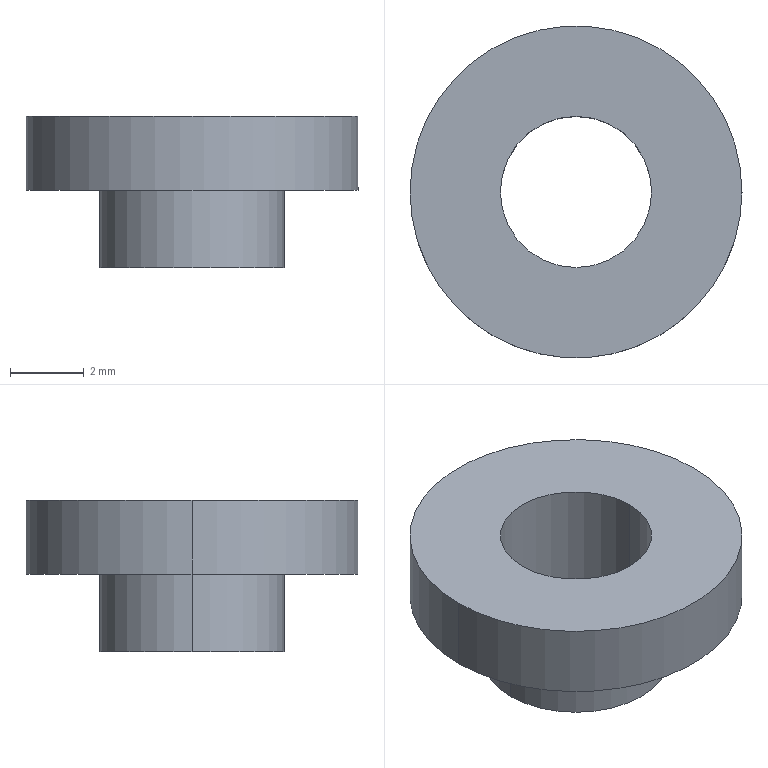Component | SolidWorks | BSH3-02-00ARubberBlankingAssembly2-1_BSH3-02-09Gasket-1 | 1 solid | 9 faces | box 9 x 9 x 4.1 mm | volume 114 mm3 | cylinder 6 | plane 3 | commonest cylinder face diameters 9 x2 5 x2 4.1 x2
build123d program:
from build123d import *


with BuildPart() as part:
    # Sketch1 → Revolve1 (revolve)
    with BuildSketch(Plane.XY, mode=Mode.PRIVATE) as revolve1_sk:
        Polygon((2.05, 0), (2.05, 4.1), (2.5, 4.1), (2.5, 2), (4.5, 2), (4.5, 0), align=None)
    revolve(revolve1_sk.sketch.rotate(Axis((0, 0, 0), (0, 1, 0)), 90), axis=Axis((0, 0, 0), (0, 1, 0)))


solid = part.part

# Placed as in the assembly
solid = solid.moved(Location((85.629, 20.762, -3.139), (-90, 0, 0)))
STEP:
#1=CARTESIAN_POINT('',(3.548,0.8174,-0.2023));
#2=VERTEX_POINT('',#1);
#3=CARTESIAN_POINT('',(3.194,0.8174,-0.2023));
#4=VERTEX_POINT('',#3);
#5=CARTESIAN_POINT('',(3.371,0.8174,-0.2023));
#6=DIRECTION('',(0.,0.,1.));
#7=DIRECTION('',(1.,0.,0.));
#8=AXIS2_PLACEMENT_3D('',#5,#6,#7);
#9=CIRCLE('',#8,0.1772);
#10=EDGE_CURVE('',#2,#4,#9,.T.);
#11=ORIENTED_EDGE('',*,*,#10,.T.);
#12=CARTESIAN_POINT('',(3.194,0.8174,-0.1236));
#13=VERTEX_POINT('',#12);
#14=CARTESIAN_POINT('',(3.194,0.8174,-0.1236));
#15=DIRECTION('',(0.,0.,1.));
#16=VECTOR('',#15,39.37);
#17=LINE('',#14,#16);
#18=EDGE_CURVE('',#4,#13,#17,.T.);
#19=ORIENTED_EDGE('',*,*,#18,.T.);
#20=CARTESIAN_POINT('',(3.548,0.8174,-0.1236));
#21=VERTEX_POINT('',#20);
#22=CARTESIAN_POINT('',(3.371,0.8174,-0.1236));
#23=DIRECTION('',(0.,0.,1.));
#24=DIRECTION('',(1.,0.,0.));
#25=AXIS2_PLACEMENT_3D('',#22,#23,#24);
#26=CIRCLE('',#25,0.1772);
#27=EDGE_CURVE('',#21,#13,#26,.T.);
#28=ORIENTED_EDGE('',*,*,#27,.F.);
#29=CARTESIAN_POINT('',(3.548,0.8174,-0.1236));
#30=DIRECTION('',(0.,0.,1.));
#31=VECTOR('',#30,39.37);
#32=LINE('',#29,#31);
#33=EDGE_CURVE('',#2,#21,#32,.T.);
#34=ORIENTED_EDGE('',*,*,#33,.F.);
#35=EDGE_LOOP('',(#11,#19,#28,#34));
#36=FACE_OUTER_BOUND('',#35,.T.);
#37=CARTESIAN_POINT('',(3.371,0.8174,-0.1236));
#38=DIRECTION('',(0.,0.,1.));
#39=DIRECTION('',(1.,0.,0.));
#40=AXIS2_PLACEMENT_3D('',#37,#38,#39);
#41=CYLINDRICAL_SURFACE('',#40,0.1772);
#42=ADVANCED_FACE('',(#36),#41,.T.);
#43=CARTESIAN_POINT('',(3.47,0.8174,-0.285));
#44=VERTEX_POINT('',#43);
#45=CARTESIAN_POINT('',(3.273,0.8174,-0.285));
#46=VERTEX_POINT('',#45);
#47=CARTESIAN_POINT('',(3.371,0.8174,-0.285));
#48=DIRECTION('',(0.,0.,1.));
#49=DIRECTION('',(1.,0.,0.));
#50=AXIS2_PLACEMENT_3D('',#47,#48,#49);
#51=CIRCLE('',#50,0.09843);
#52=EDGE_CURVE('',#44,#46,#51,.T.);
#53=ORIENTED_EDGE('',*,*,#52,.T.);
#54=CARTESIAN_POINT('',(3.273,0.8174,-0.2023));
#55=VERTEX_POINT('',#54);
#56=CARTESIAN_POINT('',(3.273,0.8174,-0.1236));
#57=DIRECTION('',(0.,0.,1.));
#58=VECTOR('',#57,39.37);
#59=LINE('',#56,#58);
#60=EDGE_CURVE('',#46,#55,#59,.T.);
#61=ORIENTED_EDGE('',*,*,#60,.T.);
#62=CARTESIAN_POINT('',(3.47,0.8174,-0.2023));
#63=VERTEX_POINT('',#62);
#64=CARTESIAN_POINT('',(3.371,0.8174,-0.2023));
#65=DIRECTION('',(0.,0.,1.));
#66=DIRECTION('',(1.,0.,0.));
#67=AXIS2_PLACEMENT_3D('',#64,#65,#66);
#68=CIRCLE('',#67,0.09843);
#69=EDGE_CURVE('',#63,#55,#68,.T.);
#70=ORIENTED_EDGE('',*,*,#69,.F.);
#71=CARTESIAN_POINT('',(3.47,0.8174,-0.1236));
#72=DIRECTION('',(0.,0.,1.));
#73=VECTOR('',#72,39.37);
#74=LINE('',#71,#73);
#75=EDGE_CURVE('',#44,#63,#74,.T.);
#76=ORIENTED_EDGE('',*,*,#75,.F.);
#77=EDGE_LOOP('',(#53,#61,#70,#76));
#78=FACE_OUTER_BOUND('',#77,.T.);
#79=CARTESIAN_POINT('',(3.371,0.8174,-0.1236));
#80=DIRECTION('',(0.,0.,1.));
#81=DIRECTION('',(1.,0.,0.));
#82=AXIS2_PLACEMENT_3D('',#79,#80,#81);
#83=CYLINDRICAL_SURFACE('',#82,0.09843);
#84=ADVANCED_FACE('',(#78),#83,.T.);
#85=CARTESIAN_POINT('',(3.291,0.8174,-0.285));
#86=VERTEX_POINT('',#85);
#87=CARTESIAN_POINT('',(3.452,0.8174,-0.285));
#88=VERTEX_POINT('',#87);
#89=CARTESIAN_POINT('',(3.371,0.8174,-0.285));
#90=DIRECTION('',(0.,0.,1.));
#91=DIRECTION('',(1.,0.,0.));
#92=AXIS2_PLACEMENT_3D('',#89,#90,#91);
#93=CIRCLE('',#92,0.08071);
#94=EDGE_CURVE('',#86,#88,#93,.T.);
#95=ORIENTED_EDGE('',*,*,#94,.F.);
#96=CARTESIAN_POINT('',(3.291,0.8174,-0.1236));
#97=VERTEX_POINT('',#96);
#98=CARTESIAN_POINT('',(3.291,0.8174,-0.1236));
#99=DIRECTION('',(0.,0.,1.));
#100=VECTOR('',#99,39.37);
#101=LINE('',#98,#100);
#102=EDGE_CURVE('',#86,#97,#101,.T.);
#103=ORIENTED_EDGE('',*,*,#102,.T.);
#104=CARTESIAN_POINT('',(3.452,0.8174,-0.1236));
#105=VERTEX_POINT('',#104);
#106=CARTESIAN_POINT('',(3.371,0.8174,-0.1236));
#107=DIRECTION('',(0.,0.,1.));
#108=DIRECTION('',(1.,0.,0.));
#109=AXIS2_PLACEMENT_3D('',#106,#107,#108);
#110=CIRCLE('',#109,0.08071);
#111=EDGE_CURVE('',#97,#105,#110,.T.);
#112=ORIENTED_EDGE('',*,*,#111,.T.);
#113=CARTESIAN_POINT('',(3.452,0.8174,-0.1236));
#114=DIRECTION('',(0.,0.,1.));
#115=VECTOR('',#114,39.37);
#116=LINE('',#113,#115);
#117=EDGE_CURVE('',#88,#105,#116,.T.);
#118=ORIENTED_EDGE('',*,*,#117,.F.);
#119=EDGE_LOOP('',(#95,#103,#112,#118));
#120=FACE_OUTER_BOUND('',#119,.T.);
#121=CARTESIAN_POINT('',(3.371,0.8174,-0.1236));
#122=DIRECTION('',(0.,0.,1.));
#123=DIRECTION('',(1.,0.,0.));
#124=AXIS2_PLACEMENT_3D('',#121,#122,#123);
#125=CYLINDRICAL_SURFACE('',#124,0.08071);
#126=ADVANCED_FACE('',(#120),#125,.F.);
#127=ORIENTED_EDGE('',*,*,#27,.T.);
#128=CARTESIAN_POINT('',(3.371,0.8174,-0.1236));
#129=DIRECTION('',(0.,0.,1.));
#130=DIRECTION('',(1.,0.,0.));
#131=AXIS2_PLACEMENT_3D('',#128,#129,#130);
#132=CIRCLE('',#131,0.1772);
#133=EDGE_CURVE('',#13,#21,#132,.T.);
#134=ORIENTED_EDGE('',*,*,#133,.T.);
#135=EDGE_LOOP('',(#127,#134));
#136=FACE_OUTER_BOUND('',#135,.T.);
#137=CARTESIAN_POINT('',(3.371,0.8174,-0.1236));
#138=DIRECTION('',(0.,0.,1.));
#139=DIRECTION('',(1.,0.,0.));
#140=AXIS2_PLACEMENT_3D('',#137,#138,#139);
#141=CIRCLE('',#140,0.08071);
#142=EDGE_CURVE('',#105,#97,#141,.T.);
#143=ORIENTED_EDGE('',*,*,#142,.F.);
#144=ORIENTED_EDGE('',*,*,#111,.F.);
#145=EDGE_LOOP('',(#143,#144));
#146=FACE_BOUND('',#145,.T.);
#147=CARTESIAN_POINT('',(3.371,0.9946,-0.1236));
#148=DIRECTION('',(0.,0.,1.));
#149=DIRECTION('',(1.,0.,-0.));
#150=AXIS2_PLACEMENT_3D('',#147,#148,#149);
#151=PLANE('',#150);
#152=ADVANCED_FACE('',(#136,#146),#151,.T.);
#153=ORIENTED_EDGE('',*,*,#102,.F.);
#154=CARTESIAN_POINT('',(3.371,0.8174,-0.285));
#155=DIRECTION('',(0.,0.,1.));
#156=DIRECTION('',(1.,0.,0.));
#157=AXIS2_PLACEMENT_3D('',#154,#155,#156);
#158=CIRCLE('',#157,0.08071);
#159=EDGE_CURVE('',#88,#86,#158,.T.);
#160=ORIENTED_EDGE('',*,*,#159,.F.);
#161=ORIENTED_EDGE('',*,*,#117,.T.);
#162=ORIENTED_EDGE('',*,*,#142,.T.);
#163=EDGE_LOOP('',(#153,#160,#161,#162));
#164=FACE_OUTER_BOUND('',#163,.T.);
#165=CARTESIAN_POINT('',(3.371,0.8174,-0.1236));
#166=DIRECTION('',(0.,0.,1.));
#167=DIRECTION('',(1.,0.,0.));
#168=AXIS2_PLACEMENT_3D('',#165,#166,#167);
#169=CYLINDRICAL_SURFACE('',#168,0.08071);
#170=ADVANCED_FACE('',(#164),#169,.F.);
#171=ORIENTED_EDGE('',*,*,#159,.T.);
#172=ORIENTED_EDGE('',*,*,#94,.T.);
#173=EDGE_LOOP('',(#171,#172));
#174=FACE_BOUND('',#173,.T.);
#175=ORIENTED_EDGE('',*,*,#52,.F.);
#176=CARTESIAN_POINT('',(3.371,0.8174,-0.285));
#177=DIRECTION('',(0.,0.,1.));
#178=DIRECTION('',(1.,0.,0.));
#179=AXIS2_PLACEMENT_3D('',#176,#177,#178);
#180=CIRCLE('',#179,0.09843);
#181=EDGE_CURVE('',#46,#44,#180,.T.);
#182=ORIENTED_EDGE('',*,*,#181,.F.);
#183=EDGE_LOOP('',(#175,#182));
#184=FACE_OUTER_BOUND('',#183,.T.);
#185=CARTESIAN_POINT('',(3.371,0.8981,-0.285));
#186=DIRECTION('',(-0.,-0.,-1.));
#187=DIRECTION('',(-1.,-0.,0.));
#188=AXIS2_PLACEMENT_3D('',#185,#186,#187);
#189=PLANE('',#188);
#190=ADVANCED_FACE('',(#174,#184),#189,.T.);
#191=ORIENTED_EDGE('',*,*,#60,.F.);
#192=ORIENTED_EDGE('',*,*,#181,.T.);
#193=ORIENTED_EDGE('',*,*,#75,.T.);
#194=CARTESIAN_POINT('',(3.371,0.8174,-0.2023));
#195=DIRECTION('',(0.,0.,1.));
#196=DIRECTION('',(1.,0.,0.));
#197=AXIS2_PLACEMENT_3D('',#194,#195,#196);
#198=CIRCLE('',#197,0.09843);
#199=EDGE_CURVE('',#55,#63,#198,.T.);
#200=ORIENTED_EDGE('',*,*,#199,.F.);
#201=EDGE_LOOP('',(#191,#192,#193,#200));
#202=FACE_OUTER_BOUND('',#201,.T.);
#203=CARTESIAN_POINT('',(3.371,0.8174,-0.1236));
#204=DIRECTION('',(0.,0.,1.));
#205=DIRECTION('',(1.,0.,0.));
#206=AXIS2_PLACEMENT_3D('',#203,#204,#205);
#207=CYLINDRICAL_SURFACE('',#206,0.09843);
#208=ADVANCED_FACE('',(#202),#207,.T.);
#209=ORIENTED_EDGE('',*,*,#69,.T.);
#210=ORIENTED_EDGE('',*,*,#199,.T.);
#211=EDGE_LOOP('',(#209,#210));
#212=FACE_BOUND('',#211,.T.);
#213=ORIENTED_EDGE('',*,*,#10,.F.);
#214=CARTESIAN_POINT('',(3.371,0.8174,-0.2023));
#215=DIRECTION('',(0.,0.,1.));
#216=DIRECTION('',(1.,0.,0.));
#217=AXIS2_PLACEMENT_3D('',#214,#215,#216);
#218=CIRCLE('',#217,0.1772);
#219=EDGE_CURVE('',#4,#2,#218,.T.);
#220=ORIENTED_EDGE('',*,*,#219,.F.);
#221=EDGE_LOOP('',(#213,#220));
#222=FACE_OUTER_BOUND('',#221,.T.);
#223=CARTESIAN_POINT('',(3.371,0.9158,-0.2023));
#224=DIRECTION('',(-0.,-0.,-1.));
#225=DIRECTION('',(-1.,-0.,0.));
#226=AXIS2_PLACEMENT_3D('',#223,#224,#225);
#227=PLANE('',#226);
#228=ADVANCED_FACE('',(#212,#222),#227,.T.);
#229=ORIENTED_EDGE('',*,*,#18,.F.);
#230=ORIENTED_EDGE('',*,*,#219,.T.);
#231=ORIENTED_EDGE('',*,*,#33,.T.);
#232=ORIENTED_EDGE('',*,*,#133,.F.);
#233=EDGE_LOOP('',(#229,#230,#231,#232));
#234=FACE_OUTER_BOUND('',#233,.T.);
#235=CARTESIAN_POINT('',(3.371,0.8174,-0.1236));
#236=DIRECTION('',(0.,0.,1.));
#237=DIRECTION('',(1.,0.,0.));
#238=AXIS2_PLACEMENT_3D('',#235,#236,#237);
#239=CYLINDRICAL_SURFACE('',#238,0.1772);
#240=ADVANCED_FACE('',(#234),#239,.T.);
#241=CLOSED_SHELL('',(#42,#84,#126,#152,#170,#190,#208,#228,#240));
#242=MANIFOLD_SOLID_BREP('',#241);
#243=CARTESIAN_POINT('',(0.,0.,0.));
#244=DIRECTION('',(0.,0.,1.));
#245=DIRECTION('',(1.,0.,0.));
#246=AXIS2_PLACEMENT_3D('',#243,#244,#245);
#247=(LENGTH_UNIT()NAMED_UNIT(*)SI_UNIT($,.METRE.));
#248=LENGTH_MEASURE_WITH_UNIT(LENGTH_MEASURE(0.0254),#247);
#249=DIMENSIONAL_EXPONENTS(1.,0.,0.,0.,0.,0.,0.);
#250=(CONVERSION_BASED_UNIT('',#248)LENGTH_UNIT()NAMED_UNIT(#249));
#251=UNCERTAINTY_MEASURE_WITH_UNIT(LENGTH_MEASURE(0.00001),#250,'','');
#252=(NAMED_UNIT(*)PLANE_ANGLE_UNIT()SI_UNIT($,.RADIAN.));
#253=(NAMED_UNIT(*)SI_UNIT($,.STERADIAN.)SOLID_ANGLE_UNIT());
#254=(GEOMETRIC_REPRESENTATION_CONTEXT(3)GLOBAL_UNCERTAINTY_ASSIGNED_CONTEXT((#251))GLOBAL_UNIT_ASSIGNED_CONTEXT((#250,#252,#253))REPRESENTATION_CONTEXT('',''));
#255=ADVANCED_BREP_SHAPE_REPRESENTATION('',(#242,#246),#254);
#256=COLOUR_RGB('',0.7922,0.8196,0.9333);
#257=FILL_AREA_STYLE_COLOUR('',#256);
#258=FILL_AREA_STYLE('',(#257));
#259=SURFACE_STYLE_FILL_AREA(#258);
#260=SURFACE_SIDE_STYLE('',(#259));
#261=SURFACE_STYLE_USAGE(.BOTH.,#260);
#262=PRESENTATION_STYLE_ASSIGNMENT((#261));
#263=STYLED_ITEM('',(#262),#242);
#264=PRESENTATION_LAYER_ASSIGNMENT('','',(#263));
#265=(LENGTH_UNIT()NAMED_UNIT(*)SI_UNIT($,.METRE.));
#266=LENGTH_MEASURE_WITH_UNIT(LENGTH_MEASURE(0.0254),#265);
#267=DIMENSIONAL_EXPONENTS(1.,0.,0.,0.,0.,0.,0.);
#268=(CONVERSION_BASED_UNIT('',#266)LENGTH_UNIT()NAMED_UNIT(#267));
#269=UNCERTAINTY_MEASURE_WITH_UNIT(LENGTH_MEASURE(0.00001),#268,'','');
#270=(NAMED_UNIT(*)PLANE_ANGLE_UNIT()SI_UNIT($,.RADIAN.));
#271=(NAMED_UNIT(*)SI_UNIT($,.STERADIAN.)SOLID_ANGLE_UNIT());
#272=(GEOMETRIC_REPRESENTATION_CONTEXT(3)GLOBAL_UNCERTAINTY_ASSIGNED_CONTEXT((#269))GLOBAL_UNIT_ASSIGNED_CONTEXT((#268,#270,#271))REPRESENTATION_CONTEXT('',''));
#273=MECHANICAL_DESIGN_GEOMETRIC_PRESENTATION_REPRESENTATION('',(#263),#272);